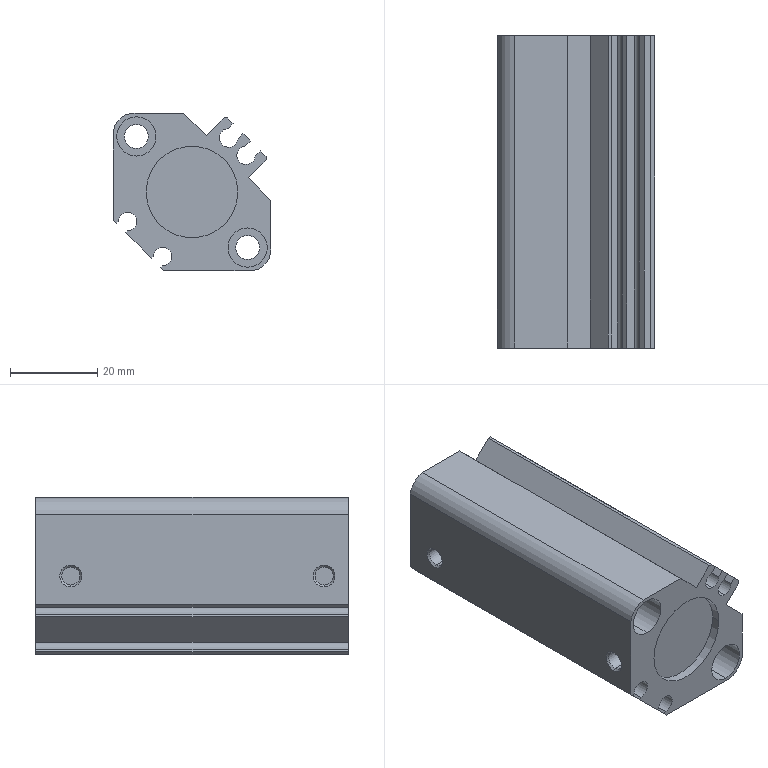Component | SolidWorks | BearingLiftingModule-1_CylinderLiftingModule-1_CDQ2B20-40DZ-L-M9B_0_0_0-1_CDQ2B20-40-L-M9B(0_0)_BODY-1 | 1 solid | 79 faces | volume 53218 mm3 | cylinder 38 | plane 37 | cone 4 | commonest cylinder face diameters 4.26 x10 9 x8 5.5 x4 4.134 x4 21 x4 10 x4 20 x2 13 x2